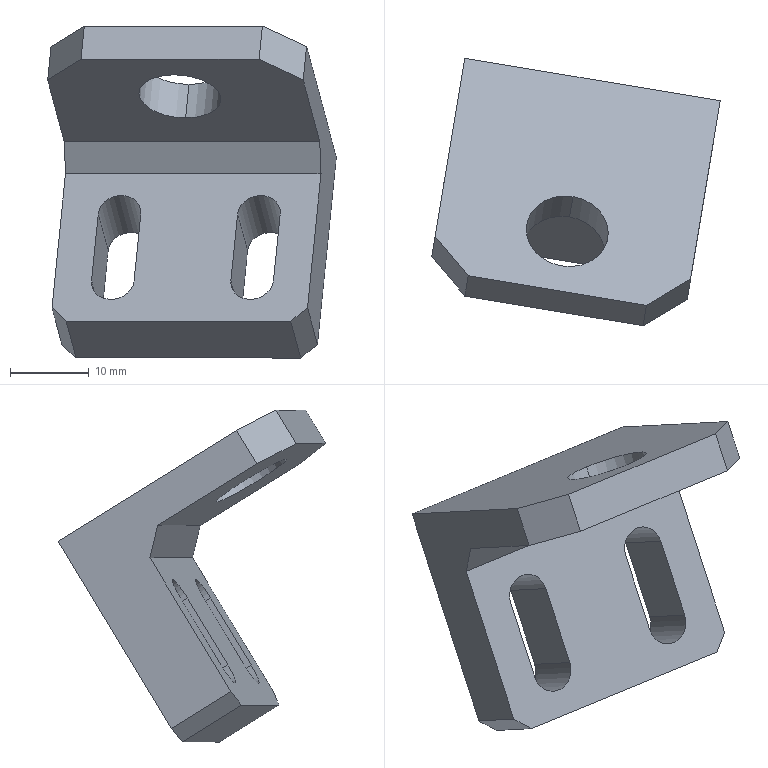Component | SolidWorks | 14AC-24-1-013-1 | 1 solid | 23 faces | box 36.76 x 34.09 x 42.29 mm | volume 10842 mm3 | plane 17 | cylinder 6 | commonest cylinder face diameters 5.5 x4 10.5 x2
build123d program:
from build123d import *

# Parameters (mm, degrees)
SKETCH1_W           = 33
SKETCH1_H           = 30
BOSS_EXTRUDE1_DEPTH = 9
SKETCH2_W           = 33
SKETCH2_H           = 5
BOSS_EXTRUDE2_DEPTH = 23
SKETCH3_R           = 5.25
CUT_EXTRUDE1_DEPTH  = 44.832
CHAMFER1_SIZE       = 5
CUT_EXTRUDE2_DEPTH  = 33.035
CHAMFER2_SIZE       = 2
CHAMFER3_SIZE       = 3


with BuildPart() as part:
    # Sketch1 → Boss-Extrude1 (new body)
    with BuildSketch(Plane.XY):
        Rectangle(SKETCH1_W, SKETCH1_H)
    extrude(amount=BOSS_EXTRUDE1_DEPTH)

    # Sketch2 → Boss-Extrude2 (add)
    with BuildSketch(Plane.XY.offset(9)):
        with Locations((0, -12.5)):
            Rectangle(SKETCH2_W, SKETCH2_H)
    extrude(amount=BOSS_EXTRUDE2_DEPTH)

    # Sketch3 → Cut-Extrude1 (cut, through all)
    with BuildSketch(Plane(origin=(0, -10, 0), x_dir=(1, 0, 0), z_dir=(0, 1, 0))):
        with Locations(Location((0, -23, 0), (0, 0, 270))):
            Circle(SKETCH3_R)
    extrude(amount=-CUT_EXTRUDE1_DEPTH, mode=Mode.SUBTRACT)

    # Chamfer1
    chamfer1_edges = [part.edges().sort_by_distance(p)[0] for p in [
        (-16.5, -12.5, 32),
        (16.5, -12.5, 32),
    ]]
    chamfer(chamfer1_edges, length=CHAMFER1_SIZE)

    # Sketch4 → Cut-Extrude2 (cut, through all)
    with BuildSketch(Plane.XY.offset(9)):
        with BuildLine():
            Line((6.25, -1), (6.25, 9))
            ThreePointArc((6.25, 9), (9, 11.75), (11.75, 9))
            Line((11.75, 9), (11.75, -1))
            ThreePointArc((11.75, -1), (9, -3.75), (6.25, -1))
        make_face()
        with BuildLine():
            Line((-11.75, -1), (-11.75, 9))
            ThreePointArc((-11.75, 9), (-9, 11.75), (-6.25, 9))
            Line((-6.25, 9), (-6.25, -1))
            ThreePointArc((-6.25, -1), (-9, -3.75), (-11.75, -1))
        make_face()
    extrude(amount=-CUT_EXTRUDE2_DEPTH, mode=Mode.SUBTRACT)

    # Chamfer2
    chamfer2_edges = [part.edges().sort_by_distance(p)[0] for p in [
        (-16.5, 15, 4.5),
        (16.5, 15, 4.5),
    ]]
    chamfer(chamfer2_edges, length=CHAMFER2_SIZE)

    # Chamfer3
    chamfer3_edges = [part.edges().sort_by_distance(p)[0] for p in [
        (0, -10, 9),
    ]]
    chamfer(chamfer3_edges, length=CHAMFER3_SIZE)


solid = part.part

# Placed as in the assembly
solid = solid.moved(Location((335.616, -100.883, -159.287), (58.173, -8.052, 175.031)))
STEP:
#1=COLOUR_RGB('',0.7922,0.8196,0.9333);
#2=FILL_AREA_STYLE_COLOUR('',#1);
#3=FILL_AREA_STYLE('',(#2));
#4=SURFACE_STYLE_FILL_AREA(#3);
#5=SURFACE_SIDE_STYLE('',(#4));
#6=SURFACE_STYLE_USAGE(.BOTH.,#5);
#7=PRESENTATION_STYLE_ASSIGNMENT((#6));
#8=CARTESIAN_POINT('',(13.166,-4.256,-5.403));
#9=VERTEX_POINT('',#8);
#10=CARTESIAN_POINT('',(13.108,-4.603,-5.187));
#11=VERTEX_POINT('',#10);
#12=CARTESIAN_POINT('',(13.137,-4.429,-5.295));
#13=DIRECTION('',(-0.08576,-0.5151,-0.8529));
#14=DIRECTION('',(-0.1401,-0.8413,0.5222));
#15=AXIS2_PLACEMENT_3D('',#12,#13,#14);
#16=CIRCLE('',#15,0.2067);
#17=EDGE_CURVE('',#9,#11,#16,.T.);
#18=ORIENTED_EDGE('',*,*,#17,.F.);
#19=CARTESIAN_POINT('',(13.149,-4.357,-5.57));
#20=VERTEX_POINT('',#19);
#21=CARTESIAN_POINT('',(13.166,-4.256,-5.403));
#22=DIRECTION('',(-0.08576,-0.5151,-0.8529));
#23=VECTOR('',#22,39.37);
#24=LINE('',#21,#23);
#25=EDGE_CURVE('',#9,#20,#24,.T.);
#26=ORIENTED_EDGE('',*,*,#25,.T.);
#27=CARTESIAN_POINT('',(13.091,-4.705,-5.355));
#28=VERTEX_POINT('',#27);
#29=CARTESIAN_POINT('',(13.12,-4.531,-5.463));
#30=DIRECTION('',(-0.08576,-0.5151,-0.8529));
#31=DIRECTION('',(-0.1401,-0.8413,0.5222));
#32=AXIS2_PLACEMENT_3D('',#29,#30,#31);
#33=CIRCLE('',#32,0.2067);
#34=EDGE_CURVE('',#20,#28,#33,.T.);
#35=ORIENTED_EDGE('',*,*,#34,.T.);
#36=CARTESIAN_POINT('',(13.108,-4.603,-5.187));
#37=DIRECTION('',(-0.08576,-0.5151,-0.8529));
#38=VECTOR('',#37,39.37);
#39=LINE('',#36,#38);
#40=EDGE_CURVE('',#11,#28,#39,.T.);
#41=ORIENTED_EDGE('',*,*,#40,.F.);
#42=EDGE_LOOP('',(#18,#26,#35,#41));
#43=FACE_OUTER_BOUND('',#42,.T.);
#44=CARTESIAN_POINT('',(13.137,-4.429,-5.295));
#45=DIRECTION('',(-0.08576,-0.5151,-0.8529));
#46=DIRECTION('',(-0.1401,-0.8413,0.5222));
#47=AXIS2_PLACEMENT_3D('',#44,#45,#46);
#48=CYLINDRICAL_SURFACE('',#47,0.2067);
#49=ADVANCED_FACE('',(#43),#48,.F.);
#50=CARTESIAN_POINT('',(12.623,-3.561,-5.768));
#51=VERTEX_POINT('',#50);
#52=CARTESIAN_POINT('',(12.529,-4.129,-6.708));
#53=VERTEX_POINT('',#52);
#54=CARTESIAN_POINT('',(12.522,-4.169,-6.775));
#55=DIRECTION('',(-0.08576,-0.5151,-0.8529));
#56=VECTOR('',#55,39.37);
#57=LINE('',#54,#56);
#58=EDGE_CURVE('',#51,#53,#57,.T.);
#59=ORIENTED_EDGE('',*,*,#58,.T.);
#60=CARTESIAN_POINT('',(12.479,-4.427,-6.523));
#61=VERTEX_POINT('',#60);
#62=CARTESIAN_POINT('',(12.479,-4.427,-6.523));
#63=DIRECTION('',(-0.1401,-0.8413,0.5222));
#64=VECTOR('',#63,39.37);
#65=LINE('',#62,#64);
#66=EDGE_CURVE('',#53,#61,#65,.T.);
#67=ORIENTED_EDGE('',*,*,#66,.T.);
#68=CARTESIAN_POINT('',(12.546,-4.021,-5.851));
#69=VERTEX_POINT('',#68);
#70=CARTESIAN_POINT('',(12.472,-4.467,-6.59));
#71=DIRECTION('',(-0.08576,-0.5151,-0.8529));
#72=VECTOR('',#71,39.37);
#73=LINE('',#70,#72);
#74=EDGE_CURVE('',#69,#61,#73,.T.);
#75=ORIENTED_EDGE('',*,*,#74,.F.);
#76=CARTESIAN_POINT('',(12.54,-4.06,-5.689));
#77=VERTEX_POINT('',#76);
#78=CARTESIAN_POINT('',(12.57,-3.88,-6.447));
#79=DIRECTION('',(-0.03841,-0.2307,0.9723));
#80=VECTOR('',#79,39.37);
#81=LINE('',#78,#80);
#82=EDGE_CURVE('',#69,#77,#81,.T.);
#83=ORIENTED_EDGE('',*,*,#82,.T.);
#84=CARTESIAN_POINT('',(12.457,-4.557,-5.38));
#85=VERTEX_POINT('',#84);
#86=CARTESIAN_POINT('',(12.43,-4.722,-5.278));
#87=DIRECTION('',(0.1401,0.8413,-0.5222));
#88=VECTOR('',#87,39.37);
#89=LINE('',#86,#88);
#90=EDGE_CURVE('',#85,#77,#89,.T.);
#91=ORIENTED_EDGE('',*,*,#90,.F.);
#92=CARTESIAN_POINT('',(12.474,-4.455,-5.212));
#93=VERTEX_POINT('',#92);
#94=CARTESIAN_POINT('',(12.373,-5.064,-6.22));
#95=DIRECTION('',(0.08576,0.5151,0.8529));
#96=VECTOR('',#95,39.37);
#97=LINE('',#94,#96);
#98=EDGE_CURVE('',#85,#93,#97,.T.);
#99=ORIENTED_EDGE('',*,*,#98,.T.);
#100=CARTESIAN_POINT('',(12.573,-3.859,-5.582));
#101=DIRECTION('',(0.1401,0.8413,-0.5222));
#102=VECTOR('',#101,39.37);
#103=LINE('',#100,#102);
#104=EDGE_CURVE('',#93,#51,#103,.T.);
#105=ORIENTED_EDGE('',*,*,#104,.T.);
#106=EDGE_LOOP('',(#59,#67,#75,#83,#91,#99,#105));
#107=FACE_OUTER_BOUND('',#106,.T.);
#108=CARTESIAN_POINT('',(12.472,-4.467,-6.59));
#109=DIRECTION('',(0.9864,-0.1642,-0.));
#110=DIRECTION('',(0.08576,0.5151,0.8529));
#111=AXIS2_PLACEMENT_3D('',#108,#109,#110);
#112=PLANE('',#111);
#113=ADVANCED_FACE('',(#107),#112,.F.);
#114=CARTESIAN_POINT('',(12.599,-4.182,-6.775));
#115=VERTEX_POINT('',#114);
#116=CARTESIAN_POINT('',(13.726,-4.37,-6.775));
#117=VERTEX_POINT('',#116);
#118=CARTESIAN_POINT('',(13.803,-4.383,-6.775));
#119=DIRECTION('',(0.9864,-0.1642,-0.));
#120=VECTOR('',#119,39.37);
#121=LINE('',#118,#120);
#122=EDGE_CURVE('',#115,#117,#121,.T.);
#123=ORIENTED_EDGE('',*,*,#122,.T.);
#124=CARTESIAN_POINT('',(13.676,-4.668,-6.59));
#125=VERTEX_POINT('',#124);
#126=CARTESIAN_POINT('',(13.676,-4.668,-6.59));
#127=DIRECTION('',(-0.1401,-0.8413,0.5222));
#128=VECTOR('',#127,39.37);
#129=LINE('',#126,#128);
#130=EDGE_CURVE('',#117,#125,#129,.T.);
#131=ORIENTED_EDGE('',*,*,#130,.T.);
#132=CARTESIAN_POINT('',(12.55,-4.48,-6.59));
#133=VERTEX_POINT('',#132);
#134=CARTESIAN_POINT('',(13.754,-4.681,-6.59));
#135=DIRECTION('',(0.9864,-0.1642,-0.));
#136=VECTOR('',#135,39.37);
#137=LINE('',#134,#136);
#138=EDGE_CURVE('',#133,#125,#137,.T.);
#139=ORIENTED_EDGE('',*,*,#138,.F.);
#140=CARTESIAN_POINT('',(12.55,-4.48,-6.59));
#141=DIRECTION('',(0.1401,0.8413,-0.5222));
#142=VECTOR('',#141,39.37);
#143=LINE('',#140,#142);
#144=EDGE_CURVE('',#133,#115,#143,.T.);
#145=ORIENTED_EDGE('',*,*,#144,.T.);
#146=EDGE_LOOP('',(#123,#131,#139,#145));
#147=FACE_OUTER_BOUND('',#146,.T.);
#148=CARTESIAN_POINT('',(13.754,-4.681,-6.59));
#149=DIRECTION('',(0.08576,0.5151,0.8529));
#150=DIRECTION('',(0.1401,0.8413,-0.5222));
#151=AXIS2_PLACEMENT_3D('',#148,#149,#150);
#152=PLANE('',#151);
#153=ADVANCED_FACE('',(#147),#152,.F.);
#154=CARTESIAN_POINT('',(13.76,-4.64,-6.523));
#155=VERTEX_POINT('',#154);
#156=CARTESIAN_POINT('',(13.828,-4.235,-5.851));
#157=VERTEX_POINT('',#156);
#158=CARTESIAN_POINT('',(13.754,-4.681,-6.59));
#159=DIRECTION('',(0.08576,0.5151,0.8529));
#160=VECTOR('',#159,39.37);
#161=LINE('',#158,#160);
#162=EDGE_CURVE('',#155,#157,#161,.T.);
#163=ORIENTED_EDGE('',*,*,#162,.F.);
#164=CARTESIAN_POINT('',(13.81,-4.342,-6.708));
#165=VERTEX_POINT('',#164);
#166=CARTESIAN_POINT('',(13.76,-4.64,-6.523));
#167=DIRECTION('',(0.1401,0.8413,-0.5222));
#168=VECTOR('',#167,39.37);
#169=LINE('',#166,#168);
#170=EDGE_CURVE('',#155,#165,#169,.T.);
#171=ORIENTED_EDGE('',*,*,#170,.T.);
#172=CARTESIAN_POINT('',(13.905,-3.774,-5.768));
#173=VERTEX_POINT('',#172);
#174=CARTESIAN_POINT('',(13.803,-4.383,-6.775));
#175=DIRECTION('',(0.08576,0.5151,0.8529));
#176=VECTOR('',#175,39.37);
#177=LINE('',#174,#176);
#178=EDGE_CURVE('',#165,#173,#177,.T.);
#179=ORIENTED_EDGE('',*,*,#178,.T.);
#180=CARTESIAN_POINT('',(13.756,-4.669,-5.212));
#181=VERTEX_POINT('',#180);
#182=CARTESIAN_POINT('',(13.855,-4.072,-5.582));
#183=DIRECTION('',(0.1401,0.8413,-0.5222));
#184=VECTOR('',#183,39.37);
#185=LINE('',#182,#184);
#186=EDGE_CURVE('',#181,#173,#185,.T.);
#187=ORIENTED_EDGE('',*,*,#186,.F.);
#188=CARTESIAN_POINT('',(13.739,-4.77,-5.38));
#189=VERTEX_POINT('',#188);
#190=CARTESIAN_POINT('',(13.654,-5.277,-6.22));
#191=DIRECTION('',(-0.08576,-0.5151,-0.8529));
#192=VECTOR('',#191,39.37);
#193=LINE('',#190,#192);
#194=EDGE_CURVE('',#181,#189,#193,.T.);
#195=ORIENTED_EDGE('',*,*,#194,.T.);
#196=CARTESIAN_POINT('',(13.822,-4.273,-5.689));
#197=VERTEX_POINT('',#196);
#198=CARTESIAN_POINT('',(13.711,-4.936,-5.278));
#199=DIRECTION('',(0.1401,0.8413,-0.5222));
#200=VECTOR('',#199,39.37);
#201=LINE('',#198,#200);
#202=EDGE_CURVE('',#189,#197,#201,.T.);
#203=ORIENTED_EDGE('',*,*,#202,.T.);
#204=CARTESIAN_POINT('',(13.852,-4.093,-6.447));
#205=DIRECTION('',(0.03841,0.2307,-0.9723));
#206=VECTOR('',#205,39.37);
#207=LINE('',#204,#206);
#208=EDGE_CURVE('',#197,#157,#207,.T.);
#209=ORIENTED_EDGE('',*,*,#208,.T.);
#210=EDGE_LOOP('',(#163,#171,#179,#187,#195,#203,#209));
#211=FACE_OUTER_BOUND('',#210,.T.);
#212=CARTESIAN_POINT('',(13.754,-4.681,-6.59));
#213=DIRECTION('',(-0.9864,0.1642,0.));
#214=DIRECTION('',(-0.08576,-0.5151,-0.8529));
#215=AXIS2_PLACEMENT_3D('',#212,#213,#214);
#216=PLANE('',#215);
#217=ADVANCED_FACE('',(#211),#216,.F.);
#218=CARTESIAN_POINT('',(13.137,-4.429,-5.295));
#219=DIRECTION('',(-0.08576,-0.5151,-0.8529));
#220=DIRECTION('',(-0.1401,-0.8413,0.5222));
#221=AXIS2_PLACEMENT_3D('',#218,#219,#220);
#222=CIRCLE('',#221,0.2067);
#223=EDGE_CURVE('',#11,#9,#222,.T.);
#224=ORIENTED_EDGE('',*,*,#223,.T.);
#225=ORIENTED_EDGE('',*,*,#17,.T.);
#226=EDGE_LOOP('',(#224,#225));
#227=FACE_BOUND('',#226,.T.);
#228=CARTESIAN_POINT('',(13.534,-4.802,-5.11));
#229=VERTEX_POINT('',#228);
#230=CARTESIAN_POINT('',(12.641,-4.653,-5.11));
#231=VERTEX_POINT('',#230);
#232=CARTESIAN_POINT('',(13.728,-4.834,-5.11));
#233=DIRECTION('',(-0.9864,0.1642,0.));
#234=VECTOR('',#233,39.37);
#235=LINE('',#232,#234);
#236=EDGE_CURVE('',#229,#231,#235,.T.);
#237=ORIENTED_EDGE('',*,*,#236,.F.);
#238=CARTESIAN_POINT('',(13.534,-4.802,-5.11));
#239=DIRECTION('',(0.7966,0.4787,-0.3692));
#240=VECTOR('',#239,39.37);
#241=LINE('',#238,#240);
#242=EDGE_CURVE('',#229,#181,#241,.T.);
#243=ORIENTED_EDGE('',*,*,#242,.T.);
#244=ORIENTED_EDGE('',*,*,#186,.T.);
#245=CARTESIAN_POINT('',(13.905,-3.774,-5.768));
#246=DIRECTION('',(-0.9864,0.1642,0.));
#247=VECTOR('',#246,39.37);
#248=LINE('',#245,#247);
#249=EDGE_CURVE('',#173,#51,#248,.T.);
#250=ORIENTED_EDGE('',*,*,#249,.T.);
#251=ORIENTED_EDGE('',*,*,#104,.F.);
#252=CARTESIAN_POINT('',(12.641,-4.653,-5.11));
#253=DIRECTION('',(0.5985,-0.711,0.3692));
#254=VECTOR('',#253,39.37);
#255=LINE('',#252,#254);
#256=EDGE_CURVE('',#93,#231,#255,.T.);
#257=ORIENTED_EDGE('',*,*,#256,.T.);
#258=EDGE_LOOP('',(#237,#243,#244,#250,#251,#257));
#259=FACE_OUTER_BOUND('',#258,.T.);
#260=CARTESIAN_POINT('',(13.855,-4.072,-5.582));
#261=DIRECTION('',(-0.08576,-0.5151,-0.8529));
#262=DIRECTION('',(-0.1401,-0.8413,0.5222));
#263=AXIS2_PLACEMENT_3D('',#260,#261,#262);
#264=PLANE('',#263);
#265=ADVANCED_FACE('',(#227,#259),#264,.F.);
#266=CARTESIAN_POINT('',(13.623,-4.326,-6.053));
#267=VERTEX_POINT('',#266);
#268=CARTESIAN_POINT('',(13.41,-4.29,-6.053));
#269=VERTEX_POINT('',#268);
#270=CARTESIAN_POINT('',(13.516,-4.308,-6.053));
#271=DIRECTION('',(-0.1401,-0.8413,0.5222));
#272=DIRECTION('',(-0.9864,0.1642,0.));
#273=AXIS2_PLACEMENT_3D('',#270,#271,#272);
#274=CIRCLE('',#273,0.1083);
#275=EDGE_CURVE('',#267,#269,#274,.T.);
#276=ORIENTED_EDGE('',*,*,#275,.F.);
#277=CARTESIAN_POINT('',(13.59,-4.528,-6.388));
#278=VERTEX_POINT('',#277);
#279=CARTESIAN_POINT('',(13.623,-4.326,-6.053));
#280=DIRECTION('',(0.08576,0.5151,0.8529));
#281=VECTOR('',#280,39.37);
#282=LINE('',#279,#281);
#283=EDGE_CURVE('',#278,#267,#282,.T.);
#284=ORIENTED_EDGE('',*,*,#283,.F.);
#285=CARTESIAN_POINT('',(13.376,-4.493,-6.388));
#286=VERTEX_POINT('',#285);
#287=CARTESIAN_POINT('',(13.483,-4.511,-6.388));
#288=DIRECTION('',(-0.1401,-0.8413,0.5222));
#289=DIRECTION('',(-0.9864,0.1642,0.));
#290=AXIS2_PLACEMENT_3D('',#287,#288,#289);
#291=CIRCLE('',#290,0.1083);
#292=EDGE_CURVE('',#286,#278,#291,.T.);
#293=ORIENTED_EDGE('',*,*,#292,.F.);
#294=CARTESIAN_POINT('',(13.41,-4.29,-6.053));
#295=DIRECTION('',(-0.08576,-0.5151,-0.8529));
#296=VECTOR('',#295,39.37);
#297=LINE('',#294,#296);
#298=EDGE_CURVE('',#269,#286,#297,.T.);
#299=ORIENTED_EDGE('',*,*,#298,.F.);
#300=EDGE_LOOP('',(#276,#284,#293,#299));
#301=FACE_BOUND('',#300,.T.);
#302=CARTESIAN_POINT('',(12.924,-4.209,-6.053));
#303=VERTEX_POINT('',#302);
#304=CARTESIAN_POINT('',(12.711,-4.174,-6.053));
#305=VERTEX_POINT('',#304);
#306=CARTESIAN_POINT('',(12.817,-4.191,-6.053));
#307=DIRECTION('',(-0.1401,-0.8413,0.5222));
#308=DIRECTION('',(-0.9864,0.1642,0.));
#309=AXIS2_PLACEMENT_3D('',#306,#307,#308);
#310=CIRCLE('',#309,0.1083);
#311=EDGE_CURVE('',#303,#305,#310,.T.);
#312=ORIENTED_EDGE('',*,*,#311,.F.);
#313=CARTESIAN_POINT('',(12.89,-4.412,-6.388));
#314=VERTEX_POINT('',#313);
#315=CARTESIAN_POINT('',(12.924,-4.209,-6.053));
#316=DIRECTION('',(0.08576,0.5151,0.8529));
#317=VECTOR('',#316,39.37);
#318=LINE('',#315,#317);
#319=EDGE_CURVE('',#314,#303,#318,.T.);
#320=ORIENTED_EDGE('',*,*,#319,.F.);
#321=CARTESIAN_POINT('',(12.677,-4.376,-6.388));
#322=VERTEX_POINT('',#321);
#323=CARTESIAN_POINT('',(12.784,-4.394,-6.388));
#324=DIRECTION('',(-0.1401,-0.8413,0.5222));
#325=DIRECTION('',(-0.9864,0.1642,0.));
#326=AXIS2_PLACEMENT_3D('',#323,#324,#325);
#327=CIRCLE('',#326,0.1083);
#328=EDGE_CURVE('',#322,#314,#327,.T.);
#329=ORIENTED_EDGE('',*,*,#328,.F.);
#330=CARTESIAN_POINT('',(12.711,-4.174,-6.053));
#331=DIRECTION('',(-0.08576,-0.5151,-0.8529));
#332=VECTOR('',#331,39.37);
#333=LINE('',#330,#332);
#334=EDGE_CURVE('',#305,#322,#333,.T.);
#335=ORIENTED_EDGE('',*,*,#334,.F.);
#336=EDGE_LOOP('',(#312,#320,#329,#335));
#337=FACE_BOUND('',#336,.T.);
#338=ORIENTED_EDGE('',*,*,#162,.T.);
#339=CARTESIAN_POINT('',(13.187,-4.128,-5.851));
#340=DIRECTION('',(-0.9864,0.1642,0.));
#341=VECTOR('',#340,39.37);
#342=LINE('',#339,#341);
#343=EDGE_CURVE('',#157,#69,#342,.T.);
#344=ORIENTED_EDGE('',*,*,#343,.T.);
#345=ORIENTED_EDGE('',*,*,#74,.T.);
#346=CARTESIAN_POINT('',(12.541,-4.474,-6.581));
#347=DIRECTION('',(0.6369,-0.4803,-0.6031));
#348=VECTOR('',#347,39.37);
#349=LINE('',#346,#348);
#350=EDGE_CURVE('',#61,#133,#349,.T.);
#351=ORIENTED_EDGE('',*,*,#350,.T.);
#352=ORIENTED_EDGE('',*,*,#138,.T.);
#353=CARTESIAN_POINT('',(13.687,-4.664,-6.581));
#354=DIRECTION('',(0.7581,0.2481,0.6031));
#355=VECTOR('',#354,39.37);
#356=LINE('',#353,#355);
#357=EDGE_CURVE('',#125,#155,#356,.T.);
#358=ORIENTED_EDGE('',*,*,#357,.T.);
#359=EDGE_LOOP('',(#338,#344,#345,#351,#352,#358));
#360=FACE_OUTER_BOUND('',#359,.T.);
#361=CARTESIAN_POINT('',(13.164,-4.27,-6.086));
#362=DIRECTION('',(-0.1401,-0.8413,0.5222));
#363=DIRECTION('',(-0.9864,0.1642,0.));
#364=AXIS2_PLACEMENT_3D('',#361,#362,#363);
#365=PLANE('',#364);
#366=ADVANCED_FACE('',(#301,#337,#360),#365,.T.);
#367=CARTESIAN_POINT('',(13.639,-4.23,-6.573));
#368=VERTEX_POINT('',#367);
#369=CARTESIAN_POINT('',(13.673,-4.027,-6.238));
#370=VERTEX_POINT('',#369);
#371=CARTESIAN_POINT('',(13.673,-4.027,-6.238));
#372=DIRECTION('',(0.08576,0.5151,0.8529));
#373=VECTOR('',#372,39.37);
#374=LINE('',#371,#373);
#375=EDGE_CURVE('',#368,#370,#374,.T.);
#376=ORIENTED_EDGE('',*,*,#375,.T.);
#377=CARTESIAN_POINT('',(13.459,-3.992,-6.238));
#378=VERTEX_POINT('',#377);
#379=CARTESIAN_POINT('',(13.566,-4.01,-6.238));
#380=DIRECTION('',(-0.1401,-0.8413,0.5222));
#381=DIRECTION('',(-0.9864,0.1642,0.));
#382=AXIS2_PLACEMENT_3D('',#379,#380,#381);
#383=CIRCLE('',#382,0.1083);
#384=EDGE_CURVE('',#370,#378,#383,.T.);
#385=ORIENTED_EDGE('',*,*,#384,.T.);
#386=CARTESIAN_POINT('',(13.426,-4.195,-6.573));
#387=VERTEX_POINT('',#386);
#388=CARTESIAN_POINT('',(13.459,-3.992,-6.238));
#389=DIRECTION('',(-0.08576,-0.5151,-0.8529));
#390=VECTOR('',#389,39.37);
#391=LINE('',#388,#390);
#392=EDGE_CURVE('',#378,#387,#391,.T.);
#393=ORIENTED_EDGE('',*,*,#392,.T.);
#394=CARTESIAN_POINT('',(13.532,-4.212,-6.573));
#395=DIRECTION('',(-0.1401,-0.8413,0.5222));
#396=DIRECTION('',(-0.9864,0.1642,0.));
#397=AXIS2_PLACEMENT_3D('',#394,#395,#396);
#398=CIRCLE('',#397,0.1083);
#399=EDGE_CURVE('',#387,#368,#398,.T.);
#400=ORIENTED_EDGE('',*,*,#399,.T.);
#401=EDGE_LOOP('',(#376,#385,#393,#400));
#402=FACE_BOUND('',#401,.T.);
#403=CARTESIAN_POINT('',(12.94,-4.114,-6.573));
#404=VERTEX_POINT('',#403);
#405=CARTESIAN_POINT('',(12.974,-3.911,-6.238));
#406=VERTEX_POINT('',#405);
#407=CARTESIAN_POINT('',(12.974,-3.911,-6.238));
#408=DIRECTION('',(0.08576,0.5151,0.8529));
#409=VECTOR('',#408,39.37);
#410=LINE('',#407,#409);
#411=EDGE_CURVE('',#404,#406,#410,.T.);
#412=ORIENTED_EDGE('',*,*,#411,.T.);
#413=CARTESIAN_POINT('',(12.76,-3.876,-6.238));
#414=VERTEX_POINT('',#413);
#415=CARTESIAN_POINT('',(12.867,-3.893,-6.238));
#416=DIRECTION('',(-0.1401,-0.8413,0.5222));
#417=DIRECTION('',(-0.9864,0.1642,0.));
#418=AXIS2_PLACEMENT_3D('',#415,#416,#417);
#419=CIRCLE('',#418,0.1083);
#420=EDGE_CURVE('',#406,#414,#419,.T.);
#421=ORIENTED_EDGE('',*,*,#420,.T.);
#422=CARTESIAN_POINT('',(12.727,-4.078,-6.573));
#423=VERTEX_POINT('',#422);
#424=CARTESIAN_POINT('',(12.76,-3.876,-6.238));
#425=DIRECTION('',(-0.08576,-0.5151,-0.8529));
#426=VECTOR('',#425,39.37);
#427=LINE('',#424,#426);
#428=EDGE_CURVE('',#414,#423,#427,.T.);
#429=ORIENTED_EDGE('',*,*,#428,.T.);
#430=CARTESIAN_POINT('',(12.833,-4.096,-6.573));
#431=DIRECTION('',(-0.1401,-0.8413,0.5222));
#432=DIRECTION('',(-0.9864,0.1642,0.));
#433=AXIS2_PLACEMENT_3D('',#430,#431,#432);
#434=CIRCLE('',#433,0.1083);
#435=EDGE_CURVE('',#423,#404,#434,.T.);
#436=ORIENTED_EDGE('',*,*,#435,.T.);
#437=EDGE_LOOP('',(#412,#421,#429,#436));
#438=FACE_BOUND('',#437,.T.);
#439=ORIENTED_EDGE('',*,*,#178,.F.);
#440=CARTESIAN_POINT('',(13.81,-4.342,-6.708));
#441=DIRECTION('',(-0.7581,-0.2481,-0.6031));
#442=VECTOR('',#441,39.37);
#443=LINE('',#440,#442);
#444=EDGE_CURVE('',#165,#117,#443,.T.);
#445=ORIENTED_EDGE('',*,*,#444,.T.);
#446=ORIENTED_EDGE('',*,*,#122,.F.);
#447=CARTESIAN_POINT('',(12.599,-4.182,-6.775));
#448=DIRECTION('',(-0.6369,0.4803,0.6031));
#449=VECTOR('',#448,39.37);
#450=LINE('',#447,#449);
#451=EDGE_CURVE('',#115,#53,#450,.T.);
#452=ORIENTED_EDGE('',*,*,#451,.T.);
#453=ORIENTED_EDGE('',*,*,#58,.F.);
#454=ORIENTED_EDGE('',*,*,#249,.F.);
#455=EDGE_LOOP('',(#439,#445,#446,#452,#453,#454));
#456=FACE_OUTER_BOUND('',#455,.T.);
#457=CARTESIAN_POINT('',(13.213,-3.972,-6.271));
#458=DIRECTION('',(-0.1401,-0.8413,0.5222));
#459=DIRECTION('',(-0.9864,0.1642,0.));
#460=AXIS2_PLACEMENT_3D('',#457,#458,#459);
#461=PLANE('',#460);
#462=ADVANCED_FACE('',(#402,#438,#456),#461,.F.);
#463=CARTESIAN_POINT('',(13.12,-4.531,-5.463));
#464=DIRECTION('',(-0.08576,-0.5151,-0.8529));
#465=DIRECTION('',(-0.1401,-0.8413,0.5222));
#466=AXIS2_PLACEMENT_3D('',#463,#464,#465);
#467=CIRCLE('',#466,0.2067);
#468=EDGE_CURVE('',#28,#20,#467,.T.);
#469=ORIENTED_EDGE('',*,*,#468,.F.);
#470=ORIENTED_EDGE('',*,*,#34,.F.);
#471=EDGE_LOOP('',(#469,#470));
#472=FACE_BOUND('',#471,.T.);
#473=ORIENTED_EDGE('',*,*,#90,.T.);
#474=CARTESIAN_POINT('',(13.822,-4.273,-5.689));
#475=DIRECTION('',(0.9864,-0.1642,-0.));
#476=VECTOR('',#475,39.37);
#477=LINE('',#474,#476);
#478=EDGE_CURVE('',#77,#197,#477,.T.);
#479=ORIENTED_EDGE('',*,*,#478,.T.);
#480=ORIENTED_EDGE('',*,*,#202,.F.);
#481=CARTESIAN_POINT('',(13.517,-4.903,-5.278));
#482=VERTEX_POINT('',#481);
#483=CARTESIAN_POINT('',(13.517,-4.903,-5.278));
#484=DIRECTION('',(-0.7966,-0.4787,0.3692));
#485=VECTOR('',#484,39.37);
#486=LINE('',#483,#485);
#487=EDGE_CURVE('',#189,#482,#486,.T.);
#488=ORIENTED_EDGE('',*,*,#487,.T.);
#489=CARTESIAN_POINT('',(12.624,-4.755,-5.278));
#490=VERTEX_POINT('',#489);
#491=CARTESIAN_POINT('',(13.711,-4.936,-5.278));
#492=DIRECTION('',(0.9864,-0.1642,-0.));
#493=VECTOR('',#492,39.37);
#494=LINE('',#491,#493);
#495=EDGE_CURVE('',#490,#482,#494,.T.);
#496=ORIENTED_EDGE('',*,*,#495,.F.);
#497=CARTESIAN_POINT('',(12.624,-4.755,-5.278));
#498=DIRECTION('',(-0.5985,0.711,-0.3692));
#499=VECTOR('',#498,39.37);
#500=LINE('',#497,#499);
#501=EDGE_CURVE('',#490,#85,#500,.T.);
#502=ORIENTED_EDGE('',*,*,#501,.T.);
#503=EDGE_LOOP('',(#473,#479,#480,#488,#496,#502));
#504=FACE_OUTER_BOUND('',#503,.T.);
#505=CARTESIAN_POINT('',(13.711,-4.936,-5.278));
#506=DIRECTION('',(0.08576,0.5151,0.8529));
#507=DIRECTION('',(0.1401,0.8413,-0.5222));
#508=AXIS2_PLACEMENT_3D('',#505,#506,#507);
#509=PLANE('',#508);
#510=ADVANCED_FACE('',(#472,#504),#509,.F.);
#511=ORIENTED_EDGE('',*,*,#495,.T.);
#512=CARTESIAN_POINT('',(13.483,-5.106,-5.613));
#513=DIRECTION('',(0.08576,0.5151,0.8529));
#514=VECTOR('',#513,39.37);
#515=LINE('',#512,#514);
#516=EDGE_CURVE('',#482,#229,#515,.T.);
#517=ORIENTED_EDGE('',*,*,#516,.T.);
#518=ORIENTED_EDGE('',*,*,#236,.T.);
#519=CARTESIAN_POINT('',(12.59,-4.957,-5.613));
#520=DIRECTION('',(-0.08576,-0.5151,-0.8529));
#521=VECTOR('',#520,39.37);
#522=LINE('',#519,#521);
#523=EDGE_CURVE('',#231,#490,#522,.T.);
#524=ORIENTED_EDGE('',*,*,#523,.T.);
#525=EDGE_LOOP('',(#511,#517,#518,#524));
#526=FACE_OUTER_BOUND('',#525,.T.);
#527=CARTESIAN_POINT('',(13.037,-5.032,-5.613));
#528=DIRECTION('',(0.1401,0.8413,-0.5222));
#529=DIRECTION('',(0.9864,-0.1642,-0.));
#530=AXIS2_PLACEMENT_3D('',#527,#528,#529);
#531=PLANE('',#530);
#532=ADVANCED_FACE('',(#526),#531,.F.);
#533=ORIENTED_EDGE('',*,*,#25,.F.);
#534=ORIENTED_EDGE('',*,*,#223,.F.);
#535=ORIENTED_EDGE('',*,*,#40,.T.);
#536=ORIENTED_EDGE('',*,*,#468,.T.);
#537=EDGE_LOOP('',(#533,#534,#535,#536));
#538=FACE_OUTER_BOUND('',#537,.T.);
#539=CARTESIAN_POINT('',(13.137,-4.429,-5.295));
#540=DIRECTION('',(-0.08576,-0.5151,-0.8529));
#541=DIRECTION('',(-0.1401,-0.8413,0.5222));
#542=AXIS2_PLACEMENT_3D('',#539,#540,#541);
#543=CYLINDRICAL_SURFACE('',#542,0.2067);
#544=ADVANCED_FACE('',(#538),#543,.F.);
#545=ORIENTED_EDGE('',*,*,#487,.F.);
#546=ORIENTED_EDGE('',*,*,#194,.F.);
#547=ORIENTED_EDGE('',*,*,#242,.F.);
#548=ORIENTED_EDGE('',*,*,#516,.F.);
#549=EDGE_LOOP('',(#545,#546,#547,#548));
#550=FACE_OUTER_BOUND('',#549,.T.);
#551=CARTESIAN_POINT('',(13.483,-5.106,-5.613));
#552=DIRECTION('',(-0.5985,0.711,-0.3692));
#553=DIRECTION('',(0.08576,0.5151,0.8529));
#554=AXIS2_PLACEMENT_3D('',#551,#552,#553);
#555=PLANE('',#554);
#556=ADVANCED_FACE('',(#550),#555,.F.);
#557=ORIENTED_EDGE('',*,*,#256,.F.);
#558=ORIENTED_EDGE('',*,*,#98,.F.);
#559=ORIENTED_EDGE('',*,*,#501,.F.);
#560=ORIENTED_EDGE('',*,*,#523,.F.);
#561=EDGE_LOOP('',(#557,#558,#559,#560));
#562=FACE_OUTER_BOUND('',#561,.T.);
#563=CARTESIAN_POINT('',(12.59,-4.957,-5.613));
#564=DIRECTION('',(0.7966,0.4787,-0.3692));
#565=DIRECTION('',(-0.08576,-0.5151,-0.8529));
#566=AXIS2_PLACEMENT_3D('',#563,#564,#565);
#567=PLANE('',#566);
#568=ADVANCED_FACE('',(#562),#567,.F.);
#569=ORIENTED_EDGE('',*,*,#311,.T.);
#570=CARTESIAN_POINT('',(12.76,-3.876,-6.238));
#571=DIRECTION('',(-0.1401,-0.8413,0.5222));
#572=VECTOR('',#571,39.37);
#573=LINE('',#570,#572);
#574=EDGE_CURVE('',#414,#305,#573,.T.);
#575=ORIENTED_EDGE('',*,*,#574,.F.);
#576=ORIENTED_EDGE('',*,*,#420,.F.);
#577=CARTESIAN_POINT('',(12.974,-3.911,-6.238));
#578=DIRECTION('',(-0.1401,-0.8413,0.5222));
#579=VECTOR('',#578,39.37);
#580=LINE('',#577,#579);
#581=EDGE_CURVE('',#406,#303,#580,.T.);
#582=ORIENTED_EDGE('',*,*,#581,.T.);
#583=EDGE_LOOP('',(#569,#575,#576,#582));
#584=FACE_OUTER_BOUND('',#583,.T.);
#585=CARTESIAN_POINT('',(12.867,-3.893,-6.238));
#586=DIRECTION('',(-0.1401,-0.8413,0.5222));
#587=DIRECTION('',(-0.9864,0.1642,0.));
#588=AXIS2_PLACEMENT_3D('',#585,#586,#587);
#589=CYLINDRICAL_SURFACE('',#588,0.1083);
#590=ADVANCED_FACE('',(#584),#589,.F.);
#591=ORIENTED_EDGE('',*,*,#319,.T.);
#592=ORIENTED_EDGE('',*,*,#581,.F.);
#593=ORIENTED_EDGE('',*,*,#411,.F.);
#594=CARTESIAN_POINT('',(12.94,-4.114,-6.573));
#595=DIRECTION('',(-0.1401,-0.8413,0.5222));
#596=VECTOR('',#595,39.37);
#597=LINE('',#594,#596);
#598=EDGE_CURVE('',#404,#314,#597,.T.);
#599=ORIENTED_EDGE('',*,*,#598,.T.);
#600=EDGE_LOOP('',(#591,#592,#593,#599));
#601=FACE_OUTER_BOUND('',#600,.T.);
#602=CARTESIAN_POINT('',(12.974,-3.911,-6.238));
#603=DIRECTION('',(0.9864,-0.1642,-0.));
#604=DIRECTION('',(-0.1401,-0.8413,0.5222));
#605=AXIS2_PLACEMENT_3D('',#602,#603,#604);
#606=PLANE('',#605);
#607=ADVANCED_FACE('',(#601),#606,.F.);
#608=ORIENTED_EDGE('',*,*,#328,.T.);
#609=ORIENTED_EDGE('',*,*,#598,.F.);
#610=ORIENTED_EDGE('',*,*,#435,.F.);
#611=CARTESIAN_POINT('',(12.727,-4.078,-6.573));
#612=DIRECTION('',(-0.1401,-0.8413,0.5222));
#613=VECTOR('',#612,39.37);
#614=LINE('',#611,#613);
#615=EDGE_CURVE('',#423,#322,#614,.T.);
#616=ORIENTED_EDGE('',*,*,#615,.T.);
#617=EDGE_LOOP('',(#608,#609,#610,#616));
#618=FACE_OUTER_BOUND('',#617,.T.);
#619=CARTESIAN_POINT('',(12.833,-4.096,-6.573));
#620=DIRECTION('',(-0.1401,-0.8413,0.5222));
#621=DIRECTION('',(-0.9864,0.1642,0.));
#622=AXIS2_PLACEMENT_3D('',#619,#620,#621);
#623=CYLINDRICAL_SURFACE('',#622,0.1083);
#624=ADVANCED_FACE('',(#618),#623,.F.);
#625=ORIENTED_EDGE('',*,*,#334,.T.);
#626=ORIENTED_EDGE('',*,*,#615,.F.);
#627=ORIENTED_EDGE('',*,*,#428,.F.);
#628=ORIENTED_EDGE('',*,*,#574,.T.);
#629=EDGE_LOOP('',(#625,#626,#627,#628));
#630=FACE_OUTER_BOUND('',#629,.T.);
#631=CARTESIAN_POINT('',(12.76,-3.876,-6.238));
#632=DIRECTION('',(-0.9864,0.1642,0.));
#633=DIRECTION('',(0.1401,0.8413,-0.5222));
#634=AXIS2_PLACEMENT_3D('',#631,#632,#633);
#635=PLANE('',#634);
#636=ADVANCED_FACE('',(#630),#635,.F.);
#637=ORIENTED_EDGE('',*,*,#275,.T.);
#638=CARTESIAN_POINT('',(13.459,-3.992,-6.238));
#639=DIRECTION('',(-0.1401,-0.8413,0.5222));
#640=VECTOR('',#639,39.37);
#641=LINE('',#638,#640);
#642=EDGE_CURVE('',#378,#269,#641,.T.);
#643=ORIENTED_EDGE('',*,*,#642,.F.);
#644=ORIENTED_EDGE('',*,*,#384,.F.);
#645=CARTESIAN_POINT('',(13.673,-4.027,-6.238));
#646=DIRECTION('',(-0.1401,-0.8413,0.5222));
#647=VECTOR('',#646,39.37);
#648=LINE('',#645,#647);
#649=EDGE_CURVE('',#370,#267,#648,.T.);
#650=ORIENTED_EDGE('',*,*,#649,.T.);
#651=EDGE_LOOP('',(#637,#643,#644,#650));
#652=FACE_OUTER_BOUND('',#651,.T.);
#653=CARTESIAN_POINT('',(13.566,-4.01,-6.238));
#654=DIRECTION('',(-0.1401,-0.8413,0.5222));
#655=DIRECTION('',(-0.9864,0.1642,0.));
#656=AXIS2_PLACEMENT_3D('',#653,#654,#655);
#657=CYLINDRICAL_SURFACE('',#656,0.1083);
#658=ADVANCED_FACE('',(#652),#657,.F.);
#659=ORIENTED_EDGE('',*,*,#283,.T.);
#660=ORIENTED_EDGE('',*,*,#649,.F.);
#661=ORIENTED_EDGE('',*,*,#375,.F.);
#662=CARTESIAN_POINT('',(13.639,-4.23,-6.573));
#663=DIRECTION('',(-0.1401,-0.8413,0.5222));
#664=VECTOR('',#663,39.37);
#665=LINE('',#662,#664);
#666=EDGE_CURVE('',#368,#278,#665,.T.);
#667=ORIENTED_EDGE('',*,*,#666,.T.);
#668=EDGE_LOOP('',(#659,#660,#661,#667));
#669=FACE_OUTER_BOUND('',#668,.T.);
#670=CARTESIAN_POINT('',(13.673,-4.027,-6.238));
#671=DIRECTION('',(0.9864,-0.1642,-0.));
#672=DIRECTION('',(-0.1401,-0.8413,0.5222));
#673=AXIS2_PLACEMENT_3D('',#670,#671,#672);
#674=PLANE('',#673);
#675=ADVANCED_FACE('',(#669),#674,.F.);
#676=ORIENTED_EDGE('',*,*,#292,.T.);
#677=ORIENTED_EDGE('',*,*,#666,.F.);
#678=ORIENTED_EDGE('',*,*,#399,.F.);
#679=CARTESIAN_POINT('',(13.426,-4.195,-6.573));
#680=DIRECTION('',(-0.1401,-0.8413,0.5222));
#681=VECTOR('',#680,39.37);
#682=LINE('',#679,#681);
#683=EDGE_CURVE('',#387,#286,#682,.T.);
#684=ORIENTED_EDGE('',*,*,#683,.T.);
#685=EDGE_LOOP('',(#676,#677,#678,#684));
#686=FACE_OUTER_BOUND('',#685,.T.);
#687=CARTESIAN_POINT('',(13.532,-4.212,-6.573));
#688=DIRECTION('',(-0.1401,-0.8413,0.5222));
#689=DIRECTION('',(-0.9864,0.1642,0.));
#690=AXIS2_PLACEMENT_3D('',#687,#688,#689);
#691=CYLINDRICAL_SURFACE('',#690,0.1083);
#692=ADVANCED_FACE('',(#686),#691,.F.);
#693=ORIENTED_EDGE('',*,*,#298,.T.);
#694=ORIENTED_EDGE('',*,*,#683,.F.);
#695=ORIENTED_EDGE('',*,*,#392,.F.);
#696=ORIENTED_EDGE('',*,*,#642,.T.);
#697=EDGE_LOOP('',(#693,#694,#695,#696));
#698=FACE_OUTER_BOUND('',#697,.T.);
#699=CARTESIAN_POINT('',(13.459,-3.992,-6.238));
#700=DIRECTION('',(-0.9864,0.1642,0.));
#701=DIRECTION('',(0.1401,0.8413,-0.5222));
#702=AXIS2_PLACEMENT_3D('',#699,#700,#701);
#703=PLANE('',#702);
#704=ADVANCED_FACE('',(#698),#703,.F.);
#705=ORIENTED_EDGE('',*,*,#357,.F.);
#706=ORIENTED_EDGE('',*,*,#130,.F.);
#707=ORIENTED_EDGE('',*,*,#444,.F.);
#708=ORIENTED_EDGE('',*,*,#170,.F.);
#709=EDGE_LOOP('',(#705,#706,#707,#708));
#710=FACE_OUTER_BOUND('',#709,.T.);
#711=CARTESIAN_POINT('',(13.76,-4.64,-6.523));
#712=DIRECTION('',(-0.6369,0.4803,0.6031));
#713=DIRECTION('',(0.1401,0.8413,-0.5222));
#714=AXIS2_PLACEMENT_3D('',#711,#712,#713);
#715=PLANE('',#714);
#716=ADVANCED_FACE('',(#710),#715,.F.);
#717=ORIENTED_EDGE('',*,*,#350,.F.);
#718=ORIENTED_EDGE('',*,*,#66,.F.);
#719=ORIENTED_EDGE('',*,*,#451,.F.);
#720=ORIENTED_EDGE('',*,*,#144,.F.);
#721=EDGE_LOOP('',(#717,#718,#719,#720));
#722=FACE_OUTER_BOUND('',#721,.T.);
#723=CARTESIAN_POINT('',(12.55,-4.48,-6.59));
#724=DIRECTION('',(0.7581,0.2481,0.6031));
#725=DIRECTION('',(0.1401,0.8413,-0.5222));
#726=AXIS2_PLACEMENT_3D('',#723,#724,#725);
#727=PLANE('',#726);
#728=ADVANCED_FACE('',(#722),#727,.F.);
#729=ORIENTED_EDGE('',*,*,#82,.F.);
#730=ORIENTED_EDGE('',*,*,#343,.F.);
#731=ORIENTED_EDGE('',*,*,#208,.F.);
#732=ORIENTED_EDGE('',*,*,#478,.F.);
#733=EDGE_LOOP('',(#729,#730,#731,#732));
#734=FACE_OUTER_BOUND('',#733,.T.);
#735=CARTESIAN_POINT('',(13.822,-4.273,-5.689));
#736=DIRECTION('',(0.1597,0.9591,0.2338));
#737=DIRECTION('',(0.9864,-0.1642,-0.));
#738=AXIS2_PLACEMENT_3D('',#735,#736,#737);
#739=PLANE('',#738);
#740=ADVANCED_FACE('',(#734),#739,.F.);
#741=CLOSED_SHELL('',(#49,#113,#153,#217,#265,#366,#462,#510,#532,#544,#556,#568,#590,#607,#624,#636,#658,#675,#692,#704,#716,#728,#740));
#742=MANIFOLD_SOLID_BREP('',#741);
#743=STYLED_ITEM('',(#7),#742);
#744=(LENGTH_UNIT()NAMED_UNIT(*)SI_UNIT($,.METRE.));
#745=LENGTH_MEASURE_WITH_UNIT(LENGTH_MEASURE(0.0254),#744);
#746=DIMENSIONAL_EXPONENTS(1.,0.,0.,0.,0.,0.,0.);
#747=(CONVERSION_BASED_UNIT('',#745)LENGTH_UNIT()NAMED_UNIT(#746));
#748=UNCERTAINTY_MEASURE_WITH_UNIT(LENGTH_MEASURE(0.00001),#747,'','');
#749=(NAMED_UNIT(*)PLANE_ANGLE_UNIT()SI_UNIT($,.RADIAN.));
#750=(NAMED_UNIT(*)SI_UNIT($,.STERADIAN.)SOLID_ANGLE_UNIT());
#751=(GEOMETRIC_REPRESENTATION_CONTEXT(3)GLOBAL_UNCERTAINTY_ASSIGNED_CONTEXT((#748))GLOBAL_UNIT_ASSIGNED_CONTEXT((#747,#749,#750))REPRESENTATION_CONTEXT('',''));
#752=MECHANICAL_DESIGN_GEOMETRIC_PRESENTATION_REPRESENTATION('',(#743),#751);
#753=CARTESIAN_POINT('',(0.,0.,0.));
#754=DIRECTION('',(0.,0.,1.));
#755=DIRECTION('',(1.,0.,0.));
#756=AXIS2_PLACEMENT_3D('',#753,#754,#755);
#757=(LENGTH_UNIT()NAMED_UNIT(*)SI_UNIT($,.METRE.));
#758=LENGTH_MEASURE_WITH_UNIT(LENGTH_MEASURE(0.0254),#757);
#759=DIMENSIONAL_EXPONENTS(1.,0.,0.,0.,0.,0.,0.);
#760=(CONVERSION_BASED_UNIT('',#758)LENGTH_UNIT()NAMED_UNIT(#759));
#761=UNCERTAINTY_MEASURE_WITH_UNIT(LENGTH_MEASURE(0.00001),#760,'','');
#762=(NAMED_UNIT(*)PLANE_ANGLE_UNIT()SI_UNIT($,.RADIAN.));
#763=(NAMED_UNIT(*)SI_UNIT($,.STERADIAN.)SOLID_ANGLE_UNIT());
#764=(GEOMETRIC_REPRESENTATION_CONTEXT(3)GLOBAL_UNCERTAINTY_ASSIGNED_CONTEXT((#761))GLOBAL_UNIT_ASSIGNED_CONTEXT((#760,#762,#763))REPRESENTATION_CONTEXT('',''));
#765=ADVANCED_BREP_SHAPE_REPRESENTATION('',(#742,#756),#764);
#766=PRESENTATION_LAYER_ASSIGNMENT('','',(#743));